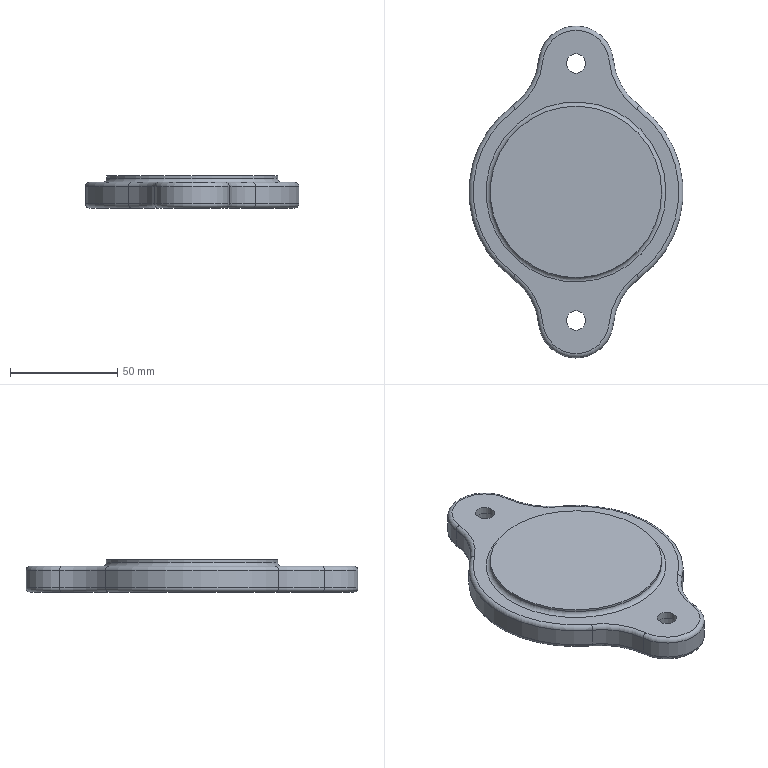Component | NX | BASE | 1 solid | 35 faces | volume 128143 mm3 | torus 17 | cylinder 13 | plane 5 | commonest cylinder face diameters 60 x4 100 x2 35 x2 9 x2 15 x2 80 x1